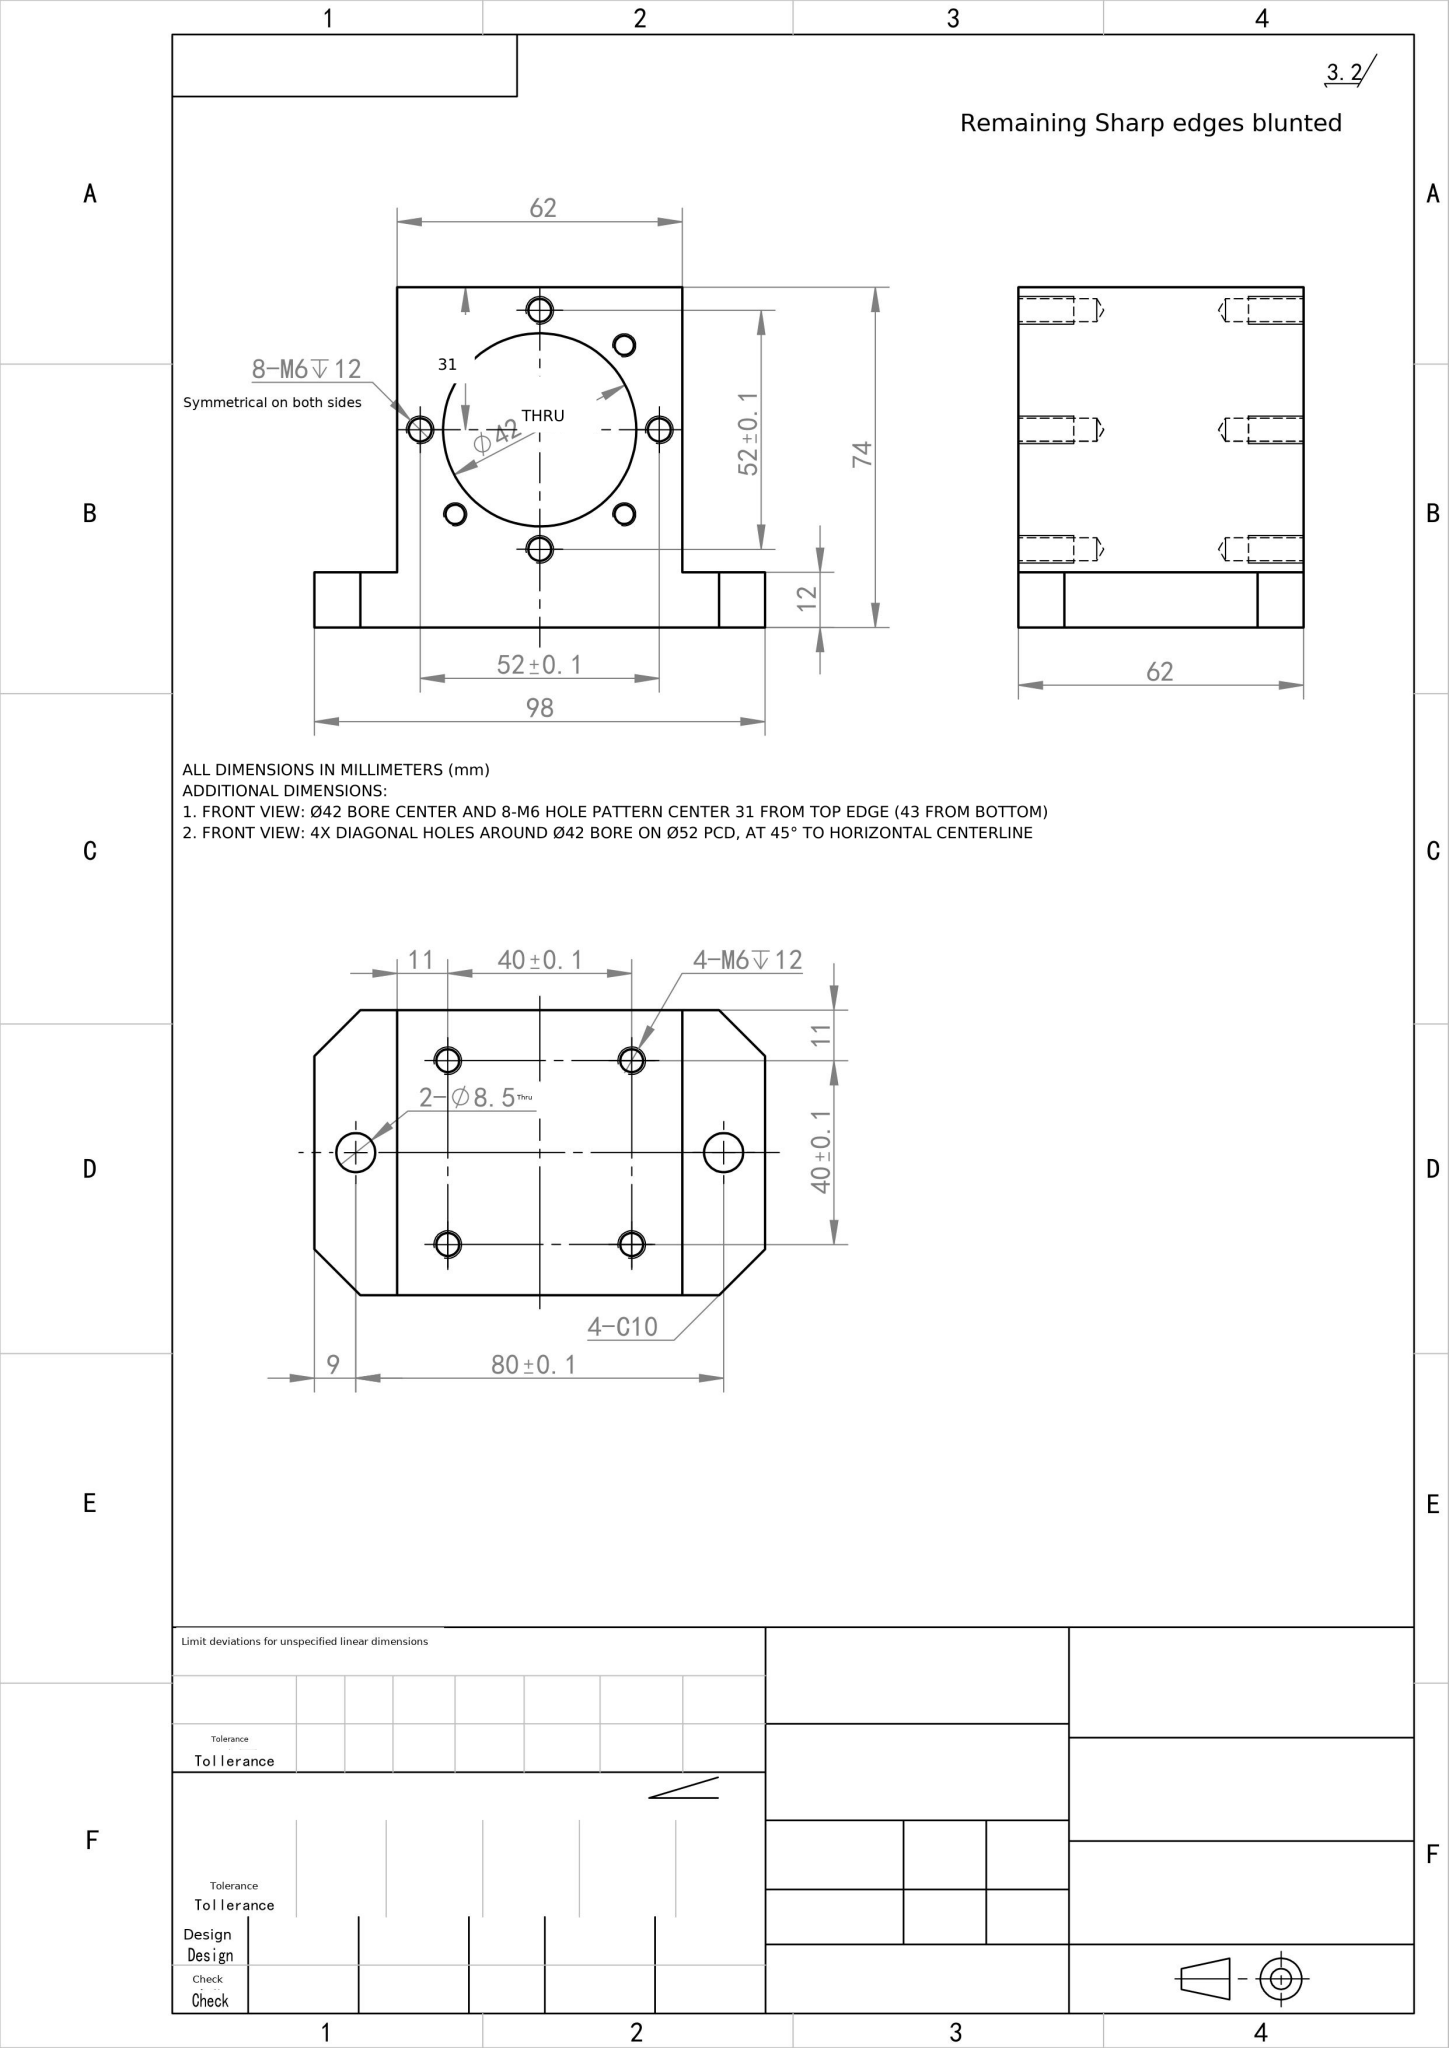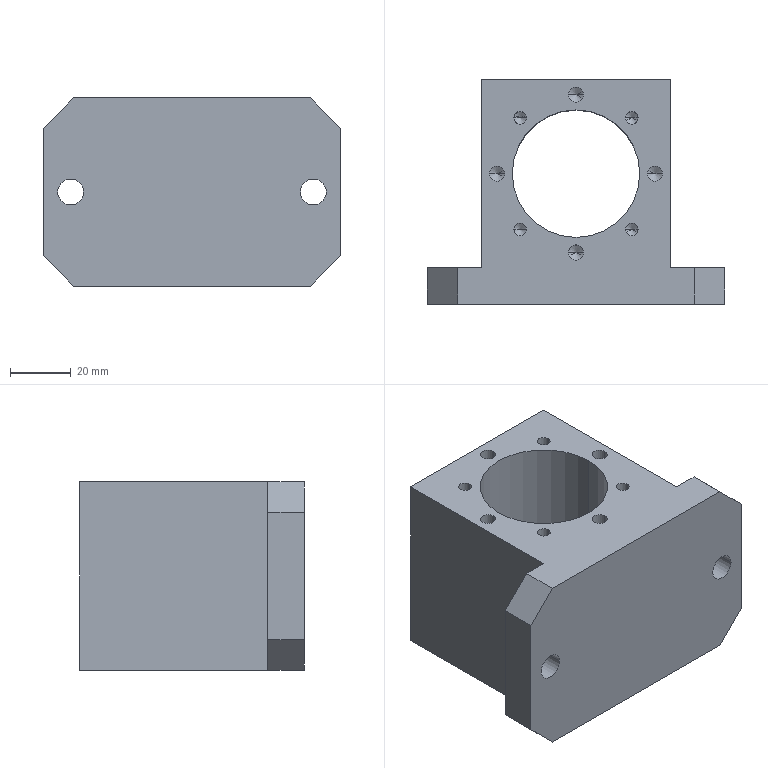Part | NX | mm | 1 solid | 104 faces | box 98 x 74 x 62 mm | volume 216026 mm3 | cylinder 50 | cone 40 | plane 14 | commonest cylinder face diameters 5 x28 4.2 x16 8.5 x4 42 x2